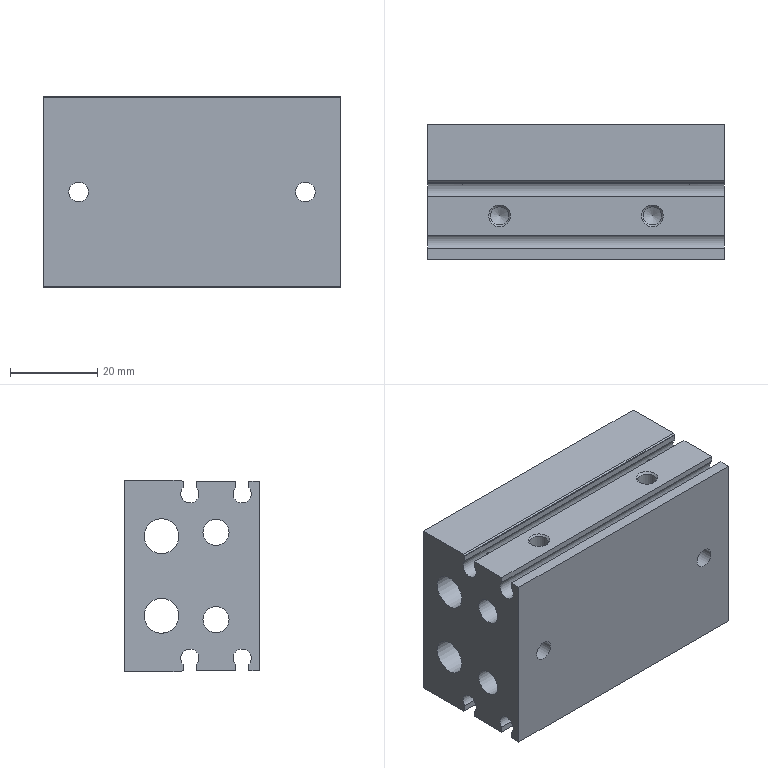Component | NX | CLAMP_CYL_1 | 1 solid | 65 faces | volume 73724 mm3 | plane 27 | cylinder 22 | cone 16 | commonest cylinder face diameters 4.2 x6 6 x6 3 x3 8 x2 4.5 x2 3.3 x2 18 x1